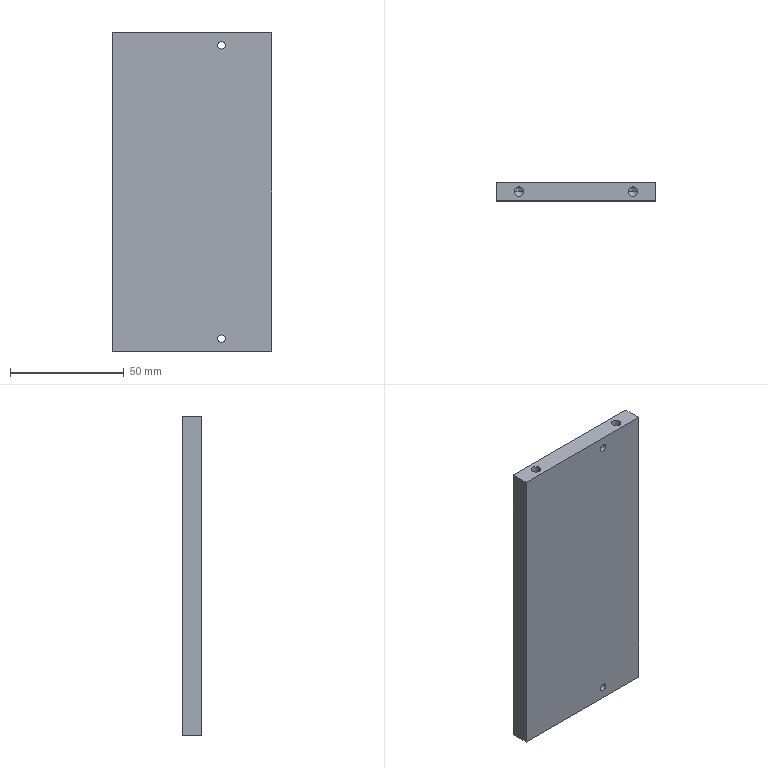Component | SolidWorks | 111.1-1 | 1 solid | 26 faces | box 70 x 8 x 140 mm | volume 77553 mm3 | cylinder 12 | cone 8 | plane 6 | commonest cylinder face diameters 4.2 x8 3.3 x4
build123d program:
from build123d import *

# Parameters (mm, degrees)
SKETCH1_W             = 140
SKETCH1_H             = 70
BOSS_EXTRUDE1_DEPTH   = 8
M5_TAPPED_HOLE1_D     = 4.2
M5_TAPPED_HOLE1_DEPTH = 12.4
M5_TAPPED_HOLE1_TIP   = 1.262
M5_TAPPED_HOLE2_D     = 4.2
M5_TAPPED_HOLE2_DEPTH = 12.4
M5_TAPPED_HOLE2_TIP   = 1.262
M4_TAPPED_HOLE1_D     = 3.3
M4_TAPPED_HOLE1_DEPTH = 10.1
M4_TAPPED_HOLE1_TIP   = 0.9914


with BuildPart() as part:
    # Sketch1 → Boss-Extrude1 (new body)
    with BuildSketch(Plane(origin=(0, 0, 0), x_dir=(1, 0, 0), z_dir=(0, 1, 0))):
        Rectangle(SKETCH1_W, SKETCH1_H)
    extrude(amount=BOSS_EXTRUDE1_DEPTH)

    # M5 Tapped Hole1
    with Locations(Plane(origin=(70, 0, 0), x_dir=(0, 0, -1), z_dir=(1, 0, 0))):
        with Locations((-25, 4), (25, 4)):
            Hole(M5_TAPPED_HOLE1_D / 2, depth=M5_TAPPED_HOLE1_DEPTH)
            with Locations((0, 0, -(M5_TAPPED_HOLE1_DEPTH + M5_TAPPED_HOLE1_TIP / 2))):  # 118° drill point
                Cone(0, M5_TAPPED_HOLE1_D / 2, M5_TAPPED_HOLE1_TIP, mode=Mode.SUBTRACT)

    # M5 Tapped Hole2
    with Locations(Plane.ZY.offset(70)):
        with Locations((-25, 4), (25, 4)):
            Hole(M5_TAPPED_HOLE2_D / 2, depth=M5_TAPPED_HOLE2_DEPTH)
            with Locations((0, 0, -(M5_TAPPED_HOLE2_DEPTH + M5_TAPPED_HOLE2_TIP / 2))):  # 118° drill point
                Cone(0, M5_TAPPED_HOLE2_D / 2, M5_TAPPED_HOLE2_TIP, mode=Mode.SUBTRACT)

    # M4 Tapped Hole1
    with Locations(Plane(origin=(0, 8, 0), x_dir=(-1, 0, 0), z_dir=(0, 1, 0))):
        with Locations((64.5, -13), (-64.5, -13)):
            Hole(M4_TAPPED_HOLE1_D / 2, depth=M4_TAPPED_HOLE1_DEPTH)
            with Locations((0, 0, -(M4_TAPPED_HOLE1_DEPTH + M4_TAPPED_HOLE1_TIP / 2))):  # 118° drill point
                Cone(0, M4_TAPPED_HOLE1_D / 2, M4_TAPPED_HOLE1_TIP, mode=Mode.SUBTRACT)


solid = part.part

# Placed as in the assembly
solid = solid.moved(Location((92, 142, 0), (0, -90, 0)))
STEP:
#1=COLOUR_RGB('',0.7922,0.8196,0.9333);
#2=FILL_AREA_STYLE_COLOUR('',#1);
#3=FILL_AREA_STYLE('',(#2));
#4=SURFACE_STYLE_FILL_AREA(#3);
#5=SURFACE_SIDE_STYLE('',(#4));
#6=SURFACE_STYLE_USAGE(.BOTH.,#5);
#7=PRESENTATION_STYLE_ASSIGNMENT((#6));
#8=CARTESIAN_POINT('',(4.199,5.591,-2.539));
#9=VERTEX_POINT('',#8);
#10=CARTESIAN_POINT('',(4.069,5.591,-2.539));
#11=VERTEX_POINT('',#10);
#12=CARTESIAN_POINT('',(4.134,5.591,-2.539));
#13=DIRECTION('',(0.,1.,0.));
#14=DIRECTION('',(-1.,0.,0.));
#15=AXIS2_PLACEMENT_3D('',#12,#13,#14);
#16=CIRCLE('',#15,0.06496);
#17=EDGE_CURVE('',#9,#11,#16,.T.);
#18=ORIENTED_EDGE('',*,*,#17,.F.);
#19=CARTESIAN_POINT('',(4.199,5.906,-2.539));
#20=VERTEX_POINT('',#19);
#21=CARTESIAN_POINT('',(4.199,5.906,-2.539));
#22=DIRECTION('',(0.,1.,0.));
#23=VECTOR('',#22,39.37);
#24=LINE('',#21,#23);
#25=EDGE_CURVE('',#9,#20,#24,.T.);
#26=ORIENTED_EDGE('',*,*,#25,.T.);
#27=CARTESIAN_POINT('',(4.069,5.906,-2.539));
#28=VERTEX_POINT('',#27);
#29=CARTESIAN_POINT('',(4.134,5.906,-2.539));
#30=DIRECTION('',(0.,1.,0.));
#31=DIRECTION('',(-1.,0.,0.));
#32=AXIS2_PLACEMENT_3D('',#29,#30,#31);
#33=CIRCLE('',#32,0.06496);
#34=EDGE_CURVE('',#20,#28,#33,.T.);
#35=ORIENTED_EDGE('',*,*,#34,.T.);
#36=CARTESIAN_POINT('',(4.069,5.906,-2.539));
#37=DIRECTION('',(0.,1.,0.));
#38=VECTOR('',#37,39.37);
#39=LINE('',#36,#38);
#40=EDGE_CURVE('',#11,#28,#39,.T.);
#41=ORIENTED_EDGE('',*,*,#40,.F.);
#42=EDGE_LOOP('',(#18,#26,#35,#41));
#43=FACE_OUTER_BOUND('',#42,.T.);
#44=CARTESIAN_POINT('',(4.134,5.906,-2.539));
#45=DIRECTION('',(0.,1.,0.));
#46=DIRECTION('',(-1.,0.,0.));
#47=AXIS2_PLACEMENT_3D('',#44,#45,#46);
#48=CYLINDRICAL_SURFACE('',#47,0.06496);
#49=ADVANCED_FACE('',(#43),#48,.F.);
#50=CARTESIAN_POINT('',(4.199,5.591,2.539));
#51=VERTEX_POINT('',#50);
#52=CARTESIAN_POINT('',(4.069,5.591,2.539));
#53=VERTEX_POINT('',#52);
#54=CARTESIAN_POINT('',(4.134,5.591,2.539));
#55=DIRECTION('',(0.,1.,0.));
#56=DIRECTION('',(-1.,0.,0.));
#57=AXIS2_PLACEMENT_3D('',#54,#55,#56);
#58=CIRCLE('',#57,0.06496);
#59=EDGE_CURVE('',#51,#53,#58,.T.);
#60=ORIENTED_EDGE('',*,*,#59,.F.);
#61=CARTESIAN_POINT('',(4.199,5.906,2.539));
#62=VERTEX_POINT('',#61);
#63=CARTESIAN_POINT('',(4.199,5.906,2.539));
#64=DIRECTION('',(0.,1.,0.));
#65=VECTOR('',#64,39.37);
#66=LINE('',#63,#65);
#67=EDGE_CURVE('',#51,#62,#66,.T.);
#68=ORIENTED_EDGE('',*,*,#67,.T.);
#69=CARTESIAN_POINT('',(4.069,5.906,2.539));
#70=VERTEX_POINT('',#69);
#71=CARTESIAN_POINT('',(4.134,5.906,2.539));
#72=DIRECTION('',(0.,1.,0.));
#73=DIRECTION('',(-1.,0.,0.));
#74=AXIS2_PLACEMENT_3D('',#71,#72,#73);
#75=CIRCLE('',#74,0.06496);
#76=EDGE_CURVE('',#62,#70,#75,.T.);
#77=ORIENTED_EDGE('',*,*,#76,.T.);
#78=CARTESIAN_POINT('',(4.069,5.906,2.539));
#79=DIRECTION('',(0.,1.,0.));
#80=VECTOR('',#79,39.37);
#81=LINE('',#78,#80);
#82=EDGE_CURVE('',#53,#70,#81,.T.);
#83=ORIENTED_EDGE('',*,*,#82,.F.);
#84=EDGE_LOOP('',(#60,#68,#77,#83));
#85=FACE_OUTER_BOUND('',#84,.T.);
#86=CARTESIAN_POINT('',(4.134,5.906,2.539));
#87=DIRECTION('',(0.,1.,0.));
#88=DIRECTION('',(-1.,0.,0.));
#89=AXIS2_PLACEMENT_3D('',#86,#87,#88);
#90=CYLINDRICAL_SURFACE('',#89,0.06496);
#91=ADVANCED_FACE('',(#85),#90,.F.);
#92=CARTESIAN_POINT('',(4.689,5.748,-2.268));
#93=VERTEX_POINT('',#92);
#94=CARTESIAN_POINT('',(4.524,5.748,-2.268));
#95=VERTEX_POINT('',#94);
#96=CARTESIAN_POINT('',(4.606,5.748,-2.268));
#97=DIRECTION('',(-0.,0.,-1.));
#98=DIRECTION('',(-1.,0.,0.));
#99=AXIS2_PLACEMENT_3D('',#96,#97,#98);
#100=CIRCLE('',#99,0.08268);
#101=EDGE_CURVE('',#93,#95,#100,.T.);
#102=ORIENTED_EDGE('',*,*,#101,.F.);
#103=CARTESIAN_POINT('',(4.689,5.748,-2.756));
#104=VERTEX_POINT('',#103);
#105=CARTESIAN_POINT('',(4.689,5.748,-2.756));
#106=DIRECTION('',(-0.,0.,-1.));
#107=VECTOR('',#106,39.37);
#108=LINE('',#105,#107);
#109=EDGE_CURVE('',#93,#104,#108,.T.);
#110=ORIENTED_EDGE('',*,*,#109,.T.);
#111=CARTESIAN_POINT('',(4.524,5.748,-2.756));
#112=VERTEX_POINT('',#111);
#113=CARTESIAN_POINT('',(4.606,5.748,-2.756));
#114=DIRECTION('',(-0.,0.,-1.));
#115=DIRECTION('',(-1.,0.,0.));
#116=AXIS2_PLACEMENT_3D('',#113,#114,#115);
#117=CIRCLE('',#116,0.08268);
#118=EDGE_CURVE('',#104,#112,#117,.T.);
#119=ORIENTED_EDGE('',*,*,#118,.T.);
#120=CARTESIAN_POINT('',(4.524,5.748,-2.756));
#121=DIRECTION('',(-0.,0.,-1.));
#122=VECTOR('',#121,39.37);
#123=LINE('',#120,#122);
#124=EDGE_CURVE('',#95,#112,#123,.T.);
#125=ORIENTED_EDGE('',*,*,#124,.F.);
#126=EDGE_LOOP('',(#102,#110,#119,#125));
#127=FACE_OUTER_BOUND('',#126,.T.);
#128=CARTESIAN_POINT('',(4.606,5.748,-2.756));
#129=DIRECTION('',(-0.,0.,-1.));
#130=DIRECTION('',(-1.,0.,0.));
#131=AXIS2_PLACEMENT_3D('',#128,#129,#130);
#132=CYLINDRICAL_SURFACE('',#131,0.08268);
#133=ADVANCED_FACE('',(#127),#132,.F.);
#134=CARTESIAN_POINT('',(4.606,5.748,-2.218));
#135=VERTEX_POINT('',#134);
#136=CARTESIAN_POINT('',(4.524,5.748,-2.268));
#137=DIRECTION('',(-0.8572,0.,-0.515));
#138=VECTOR('',#137,39.37);
#139=LINE('',#136,#138);
#140=EDGE_CURVE('',#135,#95,#139,.T.);
#141=ORIENTED_EDGE('',*,*,#140,.F.);
#142=CARTESIAN_POINT('',(4.689,5.748,-2.268));
#143=DIRECTION('',(0.8572,0.,-0.515));
#144=VECTOR('',#143,39.37);
#145=LINE('',#142,#144);
#146=EDGE_CURVE('',#135,#93,#145,.T.);
#147=ORIENTED_EDGE('',*,*,#146,.T.);
#148=ORIENTED_EDGE('',*,*,#101,.T.);
#149=EDGE_LOOP('',(#141,#147,#148));
#150=FACE_OUTER_BOUND('',#149,.T.);
#151=CARTESIAN_POINT('',(4.606,5.748,-2.268));
#152=DIRECTION('',(-0.,0.,-1.));
#153=DIRECTION('',(-1.,0.,0.));
#154=AXIS2_PLACEMENT_3D('',#151,#152,#153);
#155=CONICAL_SURFACE('',#154,0.08268,1.03);
#156=ADVANCED_FACE('',(#150),#155,.F.);
#157=CARTESIAN_POINT('',(2.72,5.748,-2.268));
#158=VERTEX_POINT('',#157);
#159=CARTESIAN_POINT('',(2.555,5.748,-2.268));
#160=VERTEX_POINT('',#159);
#161=CARTESIAN_POINT('',(2.638,5.748,-2.268));
#162=DIRECTION('',(-0.,0.,-1.));
#163=DIRECTION('',(-1.,0.,0.));
#164=AXIS2_PLACEMENT_3D('',#161,#162,#163);
#165=CIRCLE('',#164,0.08268);
#166=EDGE_CURVE('',#158,#160,#165,.T.);
#167=ORIENTED_EDGE('',*,*,#166,.F.);
#168=CARTESIAN_POINT('',(2.72,5.748,-2.756));
#169=VERTEX_POINT('',#168);
#170=CARTESIAN_POINT('',(2.72,5.748,-2.756));
#171=DIRECTION('',(-0.,0.,-1.));
#172=VECTOR('',#171,39.37);
#173=LINE('',#170,#172);
#174=EDGE_CURVE('',#158,#169,#173,.T.);
#175=ORIENTED_EDGE('',*,*,#174,.T.);
#176=CARTESIAN_POINT('',(2.555,5.748,-2.756));
#177=VERTEX_POINT('',#176);
#178=CARTESIAN_POINT('',(2.638,5.748,-2.756));
#179=DIRECTION('',(-0.,0.,-1.));
#180=DIRECTION('',(-1.,0.,0.));
#181=AXIS2_PLACEMENT_3D('',#178,#179,#180);
#182=CIRCLE('',#181,0.08268);
#183=EDGE_CURVE('',#169,#177,#182,.T.);
#184=ORIENTED_EDGE('',*,*,#183,.T.);
#185=CARTESIAN_POINT('',(2.555,5.748,-2.756));
#186=DIRECTION('',(-0.,0.,-1.));
#187=VECTOR('',#186,39.37);
#188=LINE('',#185,#187);
#189=EDGE_CURVE('',#160,#177,#188,.T.);
#190=ORIENTED_EDGE('',*,*,#189,.F.);
#191=EDGE_LOOP('',(#167,#175,#184,#190));
#192=FACE_OUTER_BOUND('',#191,.T.);
#193=CARTESIAN_POINT('',(2.638,5.748,-2.756));
#194=DIRECTION('',(-0.,0.,-1.));
#195=DIRECTION('',(-1.,0.,0.));
#196=AXIS2_PLACEMENT_3D('',#193,#194,#195);
#197=CYLINDRICAL_SURFACE('',#196,0.08268);
#198=ADVANCED_FACE('',(#192),#197,.F.);
#199=CARTESIAN_POINT('',(2.638,5.748,-2.218));
#200=VERTEX_POINT('',#199);
#201=CARTESIAN_POINT('',(2.555,5.748,-2.268));
#202=DIRECTION('',(-0.8572,0.,-0.515));
#203=VECTOR('',#202,39.37);
#204=LINE('',#201,#203);
#205=EDGE_CURVE('',#200,#160,#204,.T.);
#206=ORIENTED_EDGE('',*,*,#205,.F.);
#207=CARTESIAN_POINT('',(2.72,5.748,-2.268));
#208=DIRECTION('',(0.8572,0.,-0.515));
#209=VECTOR('',#208,39.37);
#210=LINE('',#207,#209);
#211=EDGE_CURVE('',#200,#158,#210,.T.);
#212=ORIENTED_EDGE('',*,*,#211,.T.);
#213=ORIENTED_EDGE('',*,*,#166,.T.);
#214=EDGE_LOOP('',(#206,#212,#213));
#215=FACE_OUTER_BOUND('',#214,.T.);
#216=CARTESIAN_POINT('',(2.638,5.748,-2.268));
#217=DIRECTION('',(-0.,0.,-1.));
#218=DIRECTION('',(-1.,0.,0.));
#219=AXIS2_PLACEMENT_3D('',#216,#217,#218);
#220=CONICAL_SURFACE('',#219,0.08268,1.03);
#221=ADVANCED_FACE('',(#215),#220,.F.);
#222=CARTESIAN_POINT('',(2.555,5.748,2.268));
#223=VERTEX_POINT('',#222);
#224=CARTESIAN_POINT('',(2.72,5.748,2.268));
#225=VERTEX_POINT('',#224);
#226=CARTESIAN_POINT('',(2.638,5.748,2.268));
#227=DIRECTION('',(0.,0.,1.));
#228=DIRECTION('',(1.,0.,0.));
#229=AXIS2_PLACEMENT_3D('',#226,#227,#228);
#230=CIRCLE('',#229,0.08268);
#231=EDGE_CURVE('',#223,#225,#230,.T.);
#232=ORIENTED_EDGE('',*,*,#231,.F.);
#233=CARTESIAN_POINT('',(2.555,5.748,2.756));
#234=VERTEX_POINT('',#233);
#235=CARTESIAN_POINT('',(2.555,5.748,2.756));
#236=DIRECTION('',(0.,0.,1.));
#237=VECTOR('',#236,39.37);
#238=LINE('',#235,#237);
#239=EDGE_CURVE('',#223,#234,#238,.T.);
#240=ORIENTED_EDGE('',*,*,#239,.T.);
#241=CARTESIAN_POINT('',(2.72,5.748,2.756));
#242=VERTEX_POINT('',#241);
#243=CARTESIAN_POINT('',(2.638,5.748,2.756));
#244=DIRECTION('',(0.,0.,1.));
#245=DIRECTION('',(1.,0.,0.));
#246=AXIS2_PLACEMENT_3D('',#243,#244,#245);
#247=CIRCLE('',#246,0.08268);
#248=EDGE_CURVE('',#234,#242,#247,.T.);
#249=ORIENTED_EDGE('',*,*,#248,.T.);
#250=CARTESIAN_POINT('',(2.72,5.748,2.756));
#251=DIRECTION('',(0.,0.,1.));
#252=VECTOR('',#251,39.37);
#253=LINE('',#250,#252);
#254=EDGE_CURVE('',#225,#242,#253,.T.);
#255=ORIENTED_EDGE('',*,*,#254,.F.);
#256=EDGE_LOOP('',(#232,#240,#249,#255));
#257=FACE_OUTER_BOUND('',#256,.T.);
#258=CARTESIAN_POINT('',(2.638,5.748,2.756));
#259=DIRECTION('',(0.,0.,1.));
#260=DIRECTION('',(1.,0.,0.));
#261=AXIS2_PLACEMENT_3D('',#258,#259,#260);
#262=CYLINDRICAL_SURFACE('',#261,0.08268);
#263=ADVANCED_FACE('',(#257),#262,.F.);
#264=CARTESIAN_POINT('',(2.638,5.748,2.218));
#265=VERTEX_POINT('',#264);
#266=CARTESIAN_POINT('',(2.72,5.748,2.268));
#267=DIRECTION('',(0.8572,0.,0.515));
#268=VECTOR('',#267,39.37);
#269=LINE('',#266,#268);
#270=EDGE_CURVE('',#265,#225,#269,.T.);
#271=ORIENTED_EDGE('',*,*,#270,.F.);
#272=CARTESIAN_POINT('',(2.555,5.748,2.268));
#273=DIRECTION('',(-0.8572,0.,0.515));
#274=VECTOR('',#273,39.37);
#275=LINE('',#272,#274);
#276=EDGE_CURVE('',#265,#223,#275,.T.);
#277=ORIENTED_EDGE('',*,*,#276,.T.);
#278=ORIENTED_EDGE('',*,*,#231,.T.);
#279=EDGE_LOOP('',(#271,#277,#278));
#280=FACE_OUTER_BOUND('',#279,.T.);
#281=CARTESIAN_POINT('',(2.638,5.748,2.268));
#282=DIRECTION('',(0.,0.,1.));
#283=DIRECTION('',(1.,0.,0.));
#284=AXIS2_PLACEMENT_3D('',#281,#282,#283);
#285=CONICAL_SURFACE('',#284,0.08268,1.03);
#286=ADVANCED_FACE('',(#280),#285,.F.);
#287=CARTESIAN_POINT('',(4.524,5.748,2.268));
#288=VERTEX_POINT('',#287);
#289=CARTESIAN_POINT('',(4.689,5.748,2.268));
#290=VERTEX_POINT('',#289);
#291=CARTESIAN_POINT('',(4.606,5.748,2.268));
#292=DIRECTION('',(0.,0.,1.));
#293=DIRECTION('',(1.,0.,0.));
#294=AXIS2_PLACEMENT_3D('',#291,#292,#293);
#295=CIRCLE('',#294,0.08268);
#296=EDGE_CURVE('',#288,#290,#295,.T.);
#297=ORIENTED_EDGE('',*,*,#296,.F.);
#298=CARTESIAN_POINT('',(4.524,5.748,2.756));
#299=VERTEX_POINT('',#298);
#300=CARTESIAN_POINT('',(4.524,5.748,2.756));
#301=DIRECTION('',(0.,0.,1.));
#302=VECTOR('',#301,39.37);
#303=LINE('',#300,#302);
#304=EDGE_CURVE('',#288,#299,#303,.T.);
#305=ORIENTED_EDGE('',*,*,#304,.T.);
#306=CARTESIAN_POINT('',(4.689,5.748,2.756));
#307=VERTEX_POINT('',#306);
#308=CARTESIAN_POINT('',(4.606,5.748,2.756));
#309=DIRECTION('',(0.,0.,1.));
#310=DIRECTION('',(1.,0.,0.));
#311=AXIS2_PLACEMENT_3D('',#308,#309,#310);
#312=CIRCLE('',#311,0.08268);
#313=EDGE_CURVE('',#299,#307,#312,.T.);
#314=ORIENTED_EDGE('',*,*,#313,.T.);
#315=CARTESIAN_POINT('',(4.689,5.748,2.756));
#316=DIRECTION('',(0.,0.,1.));
#317=VECTOR('',#316,39.37);
#318=LINE('',#315,#317);
#319=EDGE_CURVE('',#290,#307,#318,.T.);
#320=ORIENTED_EDGE('',*,*,#319,.F.);
#321=EDGE_LOOP('',(#297,#305,#314,#320));
#322=FACE_OUTER_BOUND('',#321,.T.);
#323=CARTESIAN_POINT('',(4.606,5.748,2.756));
#324=DIRECTION('',(0.,0.,1.));
#325=DIRECTION('',(1.,0.,0.));
#326=AXIS2_PLACEMENT_3D('',#323,#324,#325);
#327=CYLINDRICAL_SURFACE('',#326,0.08268);
#328=ADVANCED_FACE('',(#322),#327,.F.);
#329=CARTESIAN_POINT('',(4.606,5.748,2.218));
#330=VERTEX_POINT('',#329);
#331=CARTESIAN_POINT('',(4.689,5.748,2.268));
#332=DIRECTION('',(0.8572,0.,0.515));
#333=VECTOR('',#332,39.37);
#334=LINE('',#331,#333);
#335=EDGE_CURVE('',#330,#290,#334,.T.);
#336=ORIENTED_EDGE('',*,*,#335,.F.);
#337=CARTESIAN_POINT('',(4.524,5.748,2.268));
#338=DIRECTION('',(-0.8572,0.,0.515));
#339=VECTOR('',#338,39.37);
#340=LINE('',#337,#339);
#341=EDGE_CURVE('',#330,#288,#340,.T.);
#342=ORIENTED_EDGE('',*,*,#341,.T.);
#343=ORIENTED_EDGE('',*,*,#296,.T.);
#344=EDGE_LOOP('',(#336,#342,#343));
#345=FACE_OUTER_BOUND('',#344,.T.);
#346=CARTESIAN_POINT('',(4.606,5.748,2.268));
#347=DIRECTION('',(0.,0.,1.));
#348=DIRECTION('',(1.,0.,0.));
#349=AXIS2_PLACEMENT_3D('',#346,#347,#348);
#350=CONICAL_SURFACE('',#349,0.08268,1.03);
#351=ADVANCED_FACE('',(#345),#350,.F.);
#352=CARTESIAN_POINT('',(2.638,5.748,2.756));
#353=DIRECTION('',(0.,0.,1.));
#354=DIRECTION('',(1.,0.,0.));
#355=AXIS2_PLACEMENT_3D('',#352,#353,#354);
#356=CIRCLE('',#355,0.08268);
#357=EDGE_CURVE('',#242,#234,#356,.T.);
#358=ORIENTED_EDGE('',*,*,#357,.F.);
#359=ORIENTED_EDGE('',*,*,#248,.F.);
#360=EDGE_LOOP('',(#358,#359));
#361=FACE_BOUND('',#360,.T.);
#362=CARTESIAN_POINT('',(2.244,5.591,2.756));
#363=VERTEX_POINT('',#362);
#364=CARTESIAN_POINT('',(5.,5.591,2.756));
#365=VERTEX_POINT('',#364);
#366=CARTESIAN_POINT('',(5.,5.591,2.756));
#367=DIRECTION('',(1.,0.,-0.));
#368=VECTOR('',#367,39.37);
#369=LINE('',#366,#368);
#370=EDGE_CURVE('',#363,#365,#369,.T.);
#371=ORIENTED_EDGE('',*,*,#370,.T.);
#372=CARTESIAN_POINT('',(5.,5.906,2.756));
#373=VERTEX_POINT('',#372);
#374=CARTESIAN_POINT('',(5.,5.906,2.756));
#375=DIRECTION('',(0.,-1.,0.));
#376=VECTOR('',#375,39.37);
#377=LINE('',#374,#376);
#378=EDGE_CURVE('',#373,#365,#377,.T.);
#379=ORIENTED_EDGE('',*,*,#378,.F.);
#380=CARTESIAN_POINT('',(2.244,5.906,2.756));
#381=VERTEX_POINT('',#380);
#382=CARTESIAN_POINT('',(5.,5.906,2.756));
#383=DIRECTION('',(1.,0.,-0.));
#384=VECTOR('',#383,39.37);
#385=LINE('',#382,#384);
#386=EDGE_CURVE('',#381,#373,#385,.T.);
#387=ORIENTED_EDGE('',*,*,#386,.F.);
#388=CARTESIAN_POINT('',(2.244,5.906,2.756));
#389=DIRECTION('',(0.,-1.,0.));
#390=VECTOR('',#389,39.37);
#391=LINE('',#388,#390);
#392=EDGE_CURVE('',#381,#363,#391,.T.);
#393=ORIENTED_EDGE('',*,*,#392,.T.);
#394=EDGE_LOOP('',(#371,#379,#387,#393));
#395=FACE_OUTER_BOUND('',#394,.T.);
#396=CARTESIAN_POINT('',(4.606,5.748,2.756));
#397=DIRECTION('',(0.,0.,1.));
#398=DIRECTION('',(1.,0.,0.));
#399=AXIS2_PLACEMENT_3D('',#396,#397,#398);
#400=CIRCLE('',#399,0.08268);
#401=EDGE_CURVE('',#307,#299,#400,.T.);
#402=ORIENTED_EDGE('',*,*,#401,.F.);
#403=ORIENTED_EDGE('',*,*,#313,.F.);
#404=EDGE_LOOP('',(#402,#403));
#405=FACE_BOUND('',#404,.T.);
#406=CARTESIAN_POINT('',(5.,5.906,2.756));
#407=DIRECTION('',(-0.,0.,-1.));
#408=DIRECTION('',(-1.,0.,0.));
#409=AXIS2_PLACEMENT_3D('',#406,#407,#408);
#410=PLANE('',#409);
#411=ADVANCED_FACE('',(#361,#395,#405),#410,.F.);
#412=CARTESIAN_POINT('',(5.,5.591,-2.756));
#413=VERTEX_POINT('',#412);
#414=CARTESIAN_POINT('',(5.,5.591,-2.756));
#415=DIRECTION('',(0.,0.,-1.));
#416=VECTOR('',#415,39.37);
#417=LINE('',#414,#416);
#418=EDGE_CURVE('',#365,#413,#417,.T.);
#419=ORIENTED_EDGE('',*,*,#418,.T.);
#420=CARTESIAN_POINT('',(5.,5.906,-2.756));
#421=VERTEX_POINT('',#420);
#422=CARTESIAN_POINT('',(5.,5.906,-2.756));
#423=DIRECTION('',(0.,-1.,0.));
#424=VECTOR('',#423,39.37);
#425=LINE('',#422,#424);
#426=EDGE_CURVE('',#421,#413,#425,.T.);
#427=ORIENTED_EDGE('',*,*,#426,.F.);
#428=CARTESIAN_POINT('',(5.,5.906,-2.756));
#429=DIRECTION('',(0.,0.,-1.));
#430=VECTOR('',#429,39.37);
#431=LINE('',#428,#430);
#432=EDGE_CURVE('',#373,#421,#431,.T.);
#433=ORIENTED_EDGE('',*,*,#432,.F.);
#434=ORIENTED_EDGE('',*,*,#378,.T.);
#435=EDGE_LOOP('',(#419,#427,#433,#434));
#436=FACE_OUTER_BOUND('',#435,.T.);
#437=CARTESIAN_POINT('',(5.,5.906,-2.756));
#438=DIRECTION('',(-1.,0.,-0.));
#439=DIRECTION('',(-0.,0.,1.));
#440=AXIS2_PLACEMENT_3D('',#437,#438,#439);
#441=PLANE('',#440);
#442=ADVANCED_FACE('',(#436),#441,.F.);
#443=CARTESIAN_POINT('',(4.606,5.748,-2.756));
#444=DIRECTION('',(-0.,0.,-1.));
#445=DIRECTION('',(-1.,0.,0.));
#446=AXIS2_PLACEMENT_3D('',#443,#444,#445);
#447=CIRCLE('',#446,0.08268);
#448=EDGE_CURVE('',#112,#104,#447,.T.);
#449=ORIENTED_EDGE('',*,*,#448,.F.);
#450=ORIENTED_EDGE('',*,*,#118,.F.);
#451=EDGE_LOOP('',(#449,#450));
#452=FACE_BOUND('',#451,.T.);
#453=CARTESIAN_POINT('',(2.638,5.748,-2.756));
#454=DIRECTION('',(-0.,0.,-1.));
#455=DIRECTION('',(-1.,0.,0.));
#456=AXIS2_PLACEMENT_3D('',#453,#454,#455);
#457=CIRCLE('',#456,0.08268);
#458=EDGE_CURVE('',#177,#169,#457,.T.);
#459=ORIENTED_EDGE('',*,*,#458,.F.);
#460=ORIENTED_EDGE('',*,*,#183,.F.);
#461=EDGE_LOOP('',(#459,#460));
#462=FACE_BOUND('',#461,.T.);
#463=CARTESIAN_POINT('',(2.244,5.591,-2.756));
#464=VERTEX_POINT('',#463);
#465=CARTESIAN_POINT('',(5.,5.591,-2.756));
#466=DIRECTION('',(-1.,0.,0.));
#467=VECTOR('',#466,39.37);
#468=LINE('',#465,#467);
#469=EDGE_CURVE('',#413,#464,#468,.T.);
#470=ORIENTED_EDGE('',*,*,#469,.T.);
#471=CARTESIAN_POINT('',(2.244,5.906,-2.756));
#472=VERTEX_POINT('',#471);
#473=CARTESIAN_POINT('',(2.244,5.906,-2.756));
#474=DIRECTION('',(0.,-1.,0.));
#475=VECTOR('',#474,39.37);
#476=LINE('',#473,#475);
#477=EDGE_CURVE('',#472,#464,#476,.T.);
#478=ORIENTED_EDGE('',*,*,#477,.F.);
#479=CARTESIAN_POINT('',(5.,5.906,-2.756));
#480=DIRECTION('',(-1.,0.,0.));
#481=VECTOR('',#480,39.37);
#482=LINE('',#479,#481);
#483=EDGE_CURVE('',#421,#472,#482,.T.);
#484=ORIENTED_EDGE('',*,*,#483,.F.);
#485=ORIENTED_EDGE('',*,*,#426,.T.);
#486=EDGE_LOOP('',(#470,#478,#484,#485));
#487=FACE_OUTER_BOUND('',#486,.T.);
#488=CARTESIAN_POINT('',(5.,5.906,-2.756));
#489=DIRECTION('',(0.,0.,1.));
#490=DIRECTION('',(1.,0.,-0.));
#491=AXIS2_PLACEMENT_3D('',#488,#489,#490);
#492=PLANE('',#491);
#493=ADVANCED_FACE('',(#452,#462,#487),#492,.F.);
#494=CARTESIAN_POINT('',(2.244,5.591,-2.756));
#495=DIRECTION('',(-0.,0.,1.));
#496=VECTOR('',#495,39.37);
#497=LINE('',#494,#496);
#498=EDGE_CURVE('',#464,#363,#497,.T.);
#499=ORIENTED_EDGE('',*,*,#498,.T.);
#500=ORIENTED_EDGE('',*,*,#392,.F.);
#501=CARTESIAN_POINT('',(2.244,5.906,-2.756));
#502=DIRECTION('',(-0.,0.,1.));
#503=VECTOR('',#502,39.37);
#504=LINE('',#501,#503);
#505=EDGE_CURVE('',#472,#381,#504,.T.);
#506=ORIENTED_EDGE('',*,*,#505,.F.);
#507=ORIENTED_EDGE('',*,*,#477,.T.);
#508=EDGE_LOOP('',(#499,#500,#506,#507));
#509=FACE_OUTER_BOUND('',#508,.T.);
#510=CARTESIAN_POINT('',(2.244,5.906,-2.756));
#511=DIRECTION('',(1.,0.,0.));
#512=DIRECTION('',(0.,0.,-1.));
#513=AXIS2_PLACEMENT_3D('',#510,#511,#512);
#514=PLANE('',#513);
#515=ADVANCED_FACE('',(#509),#514,.F.);
#516=CARTESIAN_POINT('',(4.134,5.906,-2.539));
#517=DIRECTION('',(0.,1.,0.));
#518=DIRECTION('',(-1.,0.,0.));
#519=AXIS2_PLACEMENT_3D('',#516,#517,#518);
#520=CIRCLE('',#519,0.06496);
#521=EDGE_CURVE('',#28,#20,#520,.T.);
#522=ORIENTED_EDGE('',*,*,#521,.F.);
#523=ORIENTED_EDGE('',*,*,#34,.F.);
#524=EDGE_LOOP('',(#522,#523));
#525=FACE_BOUND('',#524,.T.);
#526=CARTESIAN_POINT('',(4.134,5.906,2.539));
#527=DIRECTION('',(0.,1.,0.));
#528=DIRECTION('',(-1.,0.,0.));
#529=AXIS2_PLACEMENT_3D('',#526,#527,#528);
#530=CIRCLE('',#529,0.06496);
#531=EDGE_CURVE('',#70,#62,#530,.T.);
#532=ORIENTED_EDGE('',*,*,#531,.F.);
#533=ORIENTED_EDGE('',*,*,#76,.F.);
#534=EDGE_LOOP('',(#532,#533));
#535=FACE_BOUND('',#534,.T.);
#536=ORIENTED_EDGE('',*,*,#386,.T.);
#537=ORIENTED_EDGE('',*,*,#432,.T.);
#538=ORIENTED_EDGE('',*,*,#483,.T.);
#539=ORIENTED_EDGE('',*,*,#505,.T.);
#540=EDGE_LOOP('',(#536,#537,#538,#539));
#541=FACE_OUTER_BOUND('',#540,.T.);
#542=CARTESIAN_POINT('',(2.244,5.906,2.756));
#543=DIRECTION('',(0.,1.,0.));
#544=DIRECTION('',(-1.,0.,-0.));
#545=AXIS2_PLACEMENT_3D('',#542,#543,#544);
#546=PLANE('',#545);
#547=ADVANCED_FACE('',(#525,#535,#541),#546,.T.);
#548=CARTESIAN_POINT('',(4.134,5.591,-2.539));
#549=DIRECTION('',(0.,1.,0.));
#550=DIRECTION('',(-1.,0.,0.));
#551=AXIS2_PLACEMENT_3D('',#548,#549,#550);
#552=CIRCLE('',#551,0.06496);
#553=EDGE_CURVE('',#11,#9,#552,.T.);
#554=ORIENTED_EDGE('',*,*,#553,.T.);
#555=ORIENTED_EDGE('',*,*,#17,.T.);
#556=EDGE_LOOP('',(#554,#555));
#557=FACE_BOUND('',#556,.T.);
#558=CARTESIAN_POINT('',(4.134,5.591,2.539));
#559=DIRECTION('',(0.,1.,0.));
#560=DIRECTION('',(-1.,0.,0.));
#561=AXIS2_PLACEMENT_3D('',#558,#559,#560);
#562=CIRCLE('',#561,0.06496);
#563=EDGE_CURVE('',#53,#51,#562,.T.);
#564=ORIENTED_EDGE('',*,*,#563,.T.);
#565=ORIENTED_EDGE('',*,*,#59,.T.);
#566=EDGE_LOOP('',(#564,#565));
#567=FACE_BOUND('',#566,.T.);
#568=ORIENTED_EDGE('',*,*,#370,.F.);
#569=ORIENTED_EDGE('',*,*,#498,.F.);
#570=ORIENTED_EDGE('',*,*,#469,.F.);
#571=ORIENTED_EDGE('',*,*,#418,.F.);
#572=EDGE_LOOP('',(#568,#569,#570,#571));
#573=FACE_OUTER_BOUND('',#572,.T.);
#574=CARTESIAN_POINT('',(2.244,5.591,2.756));
#575=DIRECTION('',(0.,1.,0.));
#576=DIRECTION('',(-1.,0.,-0.));
#577=AXIS2_PLACEMENT_3D('',#574,#575,#576);
#578=PLANE('',#577);
#579=ADVANCED_FACE('',(#557,#567,#573),#578,.F.);
#580=ORIENTED_EDGE('',*,*,#341,.F.);
#581=ORIENTED_EDGE('',*,*,#335,.T.);
#582=CARTESIAN_POINT('',(4.606,5.748,2.268));
#583=DIRECTION('',(0.,0.,1.));
#584=DIRECTION('',(1.,0.,0.));
#585=AXIS2_PLACEMENT_3D('',#582,#583,#584);
#586=CIRCLE('',#585,0.08268);
#587=EDGE_CURVE('',#290,#288,#586,.T.);
#588=ORIENTED_EDGE('',*,*,#587,.T.);
#589=EDGE_LOOP('',(#580,#581,#588));
#590=FACE_OUTER_BOUND('',#589,.T.);
#591=CARTESIAN_POINT('',(4.606,5.748,2.268));
#592=DIRECTION('',(0.,0.,1.));
#593=DIRECTION('',(1.,0.,0.));
#594=AXIS2_PLACEMENT_3D('',#591,#592,#593);
#595=CONICAL_SURFACE('',#594,0.08268,1.03);
#596=ADVANCED_FACE('',(#590),#595,.F.);
#597=ORIENTED_EDGE('',*,*,#304,.F.);
#598=ORIENTED_EDGE('',*,*,#587,.F.);
#599=ORIENTED_EDGE('',*,*,#319,.T.);
#600=ORIENTED_EDGE('',*,*,#401,.T.);
#601=EDGE_LOOP('',(#597,#598,#599,#600));
#602=FACE_OUTER_BOUND('',#601,.T.);
#603=CARTESIAN_POINT('',(4.606,5.748,2.756));
#604=DIRECTION('',(0.,0.,1.));
#605=DIRECTION('',(1.,0.,0.));
#606=AXIS2_PLACEMENT_3D('',#603,#604,#605);
#607=CYLINDRICAL_SURFACE('',#606,0.08268);
#608=ADVANCED_FACE('',(#602),#607,.F.);
#609=ORIENTED_EDGE('',*,*,#276,.F.);
#610=ORIENTED_EDGE('',*,*,#270,.T.);
#611=CARTESIAN_POINT('',(2.638,5.748,2.268));
#612=DIRECTION('',(0.,0.,1.));
#613=DIRECTION('',(1.,0.,0.));
#614=AXIS2_PLACEMENT_3D('',#611,#612,#613);
#615=CIRCLE('',#614,0.08268);
#616=EDGE_CURVE('',#225,#223,#615,.T.);
#617=ORIENTED_EDGE('',*,*,#616,.T.);
#618=EDGE_LOOP('',(#609,#610,#617));
#619=FACE_OUTER_BOUND('',#618,.T.);
#620=CARTESIAN_POINT('',(2.638,5.748,2.268));
#621=DIRECTION('',(0.,0.,1.));
#622=DIRECTION('',(1.,0.,0.));
#623=AXIS2_PLACEMENT_3D('',#620,#621,#622);
#624=CONICAL_SURFACE('',#623,0.08268,1.03);
#625=ADVANCED_FACE('',(#619),#624,.F.);
#626=ORIENTED_EDGE('',*,*,#239,.F.);
#627=ORIENTED_EDGE('',*,*,#616,.F.);
#628=ORIENTED_EDGE('',*,*,#254,.T.);
#629=ORIENTED_EDGE('',*,*,#357,.T.);
#630=EDGE_LOOP('',(#626,#627,#628,#629));
#631=FACE_OUTER_BOUND('',#630,.T.);
#632=CARTESIAN_POINT('',(2.638,5.748,2.756));
#633=DIRECTION('',(0.,0.,1.));
#634=DIRECTION('',(1.,0.,0.));
#635=AXIS2_PLACEMENT_3D('',#632,#633,#634);
#636=CYLINDRICAL_SURFACE('',#635,0.08268);
#637=ADVANCED_FACE('',(#631),#636,.F.);
#638=ORIENTED_EDGE('',*,*,#211,.F.);
#639=ORIENTED_EDGE('',*,*,#205,.T.);
#640=CARTESIAN_POINT('',(2.638,5.748,-2.268));
#641=DIRECTION('',(-0.,0.,-1.));
#642=DIRECTION('',(-1.,0.,0.));
#643=AXIS2_PLACEMENT_3D('',#640,#641,#642);
#644=CIRCLE('',#643,0.08268);
#645=EDGE_CURVE('',#160,#158,#644,.T.);
#646=ORIENTED_EDGE('',*,*,#645,.T.);
#647=EDGE_LOOP('',(#638,#639,#646));
#648=FACE_OUTER_BOUND('',#647,.T.);
#649=CARTESIAN_POINT('',(2.638,5.748,-2.268));
#650=DIRECTION('',(-0.,0.,-1.));
#651=DIRECTION('',(-1.,0.,0.));
#652=AXIS2_PLACEMENT_3D('',#649,#650,#651);
#653=CONICAL_SURFACE('',#652,0.08268,1.03);
#654=ADVANCED_FACE('',(#648),#653,.F.);
#655=ORIENTED_EDGE('',*,*,#174,.F.);
#656=ORIENTED_EDGE('',*,*,#645,.F.);
#657=ORIENTED_EDGE('',*,*,#189,.T.);
#658=ORIENTED_EDGE('',*,*,#458,.T.);
#659=EDGE_LOOP('',(#655,#656,#657,#658));
#660=FACE_OUTER_BOUND('',#659,.T.);
#661=CARTESIAN_POINT('',(2.638,5.748,-2.756));
#662=DIRECTION('',(-0.,0.,-1.));
#663=DIRECTION('',(-1.,0.,0.));
#664=AXIS2_PLACEMENT_3D('',#661,#662,#663);
#665=CYLINDRICAL_SURFACE('',#664,0.08268);
#666=ADVANCED_FACE('',(#660),#665,.F.);
#667=ORIENTED_EDGE('',*,*,#146,.F.);
#668=ORIENTED_EDGE('',*,*,#140,.T.);
#669=CARTESIAN_POINT('',(4.606,5.748,-2.268));
#670=DIRECTION('',(-0.,0.,-1.));
#671=DIRECTION('',(-1.,0.,0.));
#672=AXIS2_PLACEMENT_3D('',#669,#670,#671);
#673=CIRCLE('',#672,0.08268);
#674=EDGE_CURVE('',#95,#93,#673,.T.);
#675=ORIENTED_EDGE('',*,*,#674,.T.);
#676=EDGE_LOOP('',(#667,#668,#675));
#677=FACE_OUTER_BOUND('',#676,.T.);
#678=CARTESIAN_POINT('',(4.606,5.748,-2.268));
#679=DIRECTION('',(-0.,0.,-1.));
#680=DIRECTION('',(-1.,0.,0.));
#681=AXIS2_PLACEMENT_3D('',#678,#679,#680);
#682=CONICAL_SURFACE('',#681,0.08268,1.03);
#683=ADVANCED_FACE('',(#677),#682,.F.);
#684=ORIENTED_EDGE('',*,*,#109,.F.);
#685=ORIENTED_EDGE('',*,*,#674,.F.);
#686=ORIENTED_EDGE('',*,*,#124,.T.);
#687=ORIENTED_EDGE('',*,*,#448,.T.);
#688=EDGE_LOOP('',(#684,#685,#686,#687));
#689=FACE_OUTER_BOUND('',#688,.T.);
#690=CARTESIAN_POINT('',(4.606,5.748,-2.756));
#691=DIRECTION('',(-0.,0.,-1.));
#692=DIRECTION('',(-1.,0.,0.));
#693=AXIS2_PLACEMENT_3D('',#690,#691,#692);
#694=CYLINDRICAL_SURFACE('',#693,0.08268);
#695=ADVANCED_FACE('',(#689),#694,.F.);
#696=ORIENTED_EDGE('',*,*,#67,.F.);
#697=ORIENTED_EDGE('',*,*,#563,.F.);
#698=ORIENTED_EDGE('',*,*,#82,.T.);
#699=ORIENTED_EDGE('',*,*,#531,.T.);
#700=EDGE_LOOP('',(#696,#697,#698,#699));
#701=FACE_OUTER_BOUND('',#700,.T.);
#702=CARTESIAN_POINT('',(4.134,5.906,2.539));
#703=DIRECTION('',(0.,1.,0.));
#704=DIRECTION('',(-1.,0.,0.));
#705=AXIS2_PLACEMENT_3D('',#702,#703,#704);
#706=CYLINDRICAL_SURFACE('',#705,0.06496);
#707=ADVANCED_FACE('',(#701),#706,.F.);
#708=ORIENTED_EDGE('',*,*,#25,.F.);
#709=ORIENTED_EDGE('',*,*,#553,.F.);
#710=ORIENTED_EDGE('',*,*,#40,.T.);
#711=ORIENTED_EDGE('',*,*,#521,.T.);
#712=EDGE_LOOP('',(#708,#709,#710,#711));
#713=FACE_OUTER_BOUND('',#712,.T.);
#714=CARTESIAN_POINT('',(4.134,5.906,-2.539));
#715=DIRECTION('',(0.,1.,0.));
#716=DIRECTION('',(-1.,0.,0.));
#717=AXIS2_PLACEMENT_3D('',#714,#715,#716);
#718=CYLINDRICAL_SURFACE('',#717,0.06496);
#719=ADVANCED_FACE('',(#713),#718,.F.);
#720=CLOSED_SHELL('',(#49,#91,#133,#156,#198,#221,#263,#286,#328,#351,#411,#442,#493,#515,#547,#579,#596,#608,#625,#637,#654,#666,#683,#695,#707,#719));
#721=MANIFOLD_SOLID_BREP('',#720);
#722=STYLED_ITEM('',(#7),#721);
#723=PRESENTATION_LAYER_ASSIGNMENT('','',(#722));
#724=CARTESIAN_POINT('',(0.,0.,0.));
#725=DIRECTION('',(0.,0.,1.));
#726=DIRECTION('',(1.,0.,0.));
#727=AXIS2_PLACEMENT_3D('',#724,#725,#726);
#728=(LENGTH_UNIT()NAMED_UNIT(*)SI_UNIT($,.METRE.));
#729=LENGTH_MEASURE_WITH_UNIT(LENGTH_MEASURE(0.0254),#728);
#730=DIMENSIONAL_EXPONENTS(1.,0.,0.,0.,0.,0.,0.);
#731=(CONVERSION_BASED_UNIT('',#729)LENGTH_UNIT()NAMED_UNIT(#730));
#732=UNCERTAINTY_MEASURE_WITH_UNIT(LENGTH_MEASURE(0.00001),#731,'','');
#733=(NAMED_UNIT(*)PLANE_ANGLE_UNIT()SI_UNIT($,.RADIAN.));
#734=(NAMED_UNIT(*)SI_UNIT($,.STERADIAN.)SOLID_ANGLE_UNIT());
#735=(GEOMETRIC_REPRESENTATION_CONTEXT(3)GLOBAL_UNCERTAINTY_ASSIGNED_CONTEXT((#732))GLOBAL_UNIT_ASSIGNED_CONTEXT((#731,#733,#734))REPRESENTATION_CONTEXT('',''));
#736=ADVANCED_BREP_SHAPE_REPRESENTATION('',(#721,#727),#735);
#737=(LENGTH_UNIT()NAMED_UNIT(*)SI_UNIT($,.METRE.));
#738=LENGTH_MEASURE_WITH_UNIT(LENGTH_MEASURE(0.0254),#737);
#739=DIMENSIONAL_EXPONENTS(1.,0.,0.,0.,0.,0.,0.);
#740=(CONVERSION_BASED_UNIT('',#738)LENGTH_UNIT()NAMED_UNIT(#739));
#741=UNCERTAINTY_MEASURE_WITH_UNIT(LENGTH_MEASURE(0.00001),#740,'','');
#742=(NAMED_UNIT(*)PLANE_ANGLE_UNIT()SI_UNIT($,.RADIAN.));
#743=(NAMED_UNIT(*)SI_UNIT($,.STERADIAN.)SOLID_ANGLE_UNIT());
#744=(GEOMETRIC_REPRESENTATION_CONTEXT(3)GLOBAL_UNCERTAINTY_ASSIGNED_CONTEXT((#741))GLOBAL_UNIT_ASSIGNED_CONTEXT((#740,#742,#743))REPRESENTATION_CONTEXT('',''));
#745=MECHANICAL_DESIGN_GEOMETRIC_PRESENTATION_REPRESENTATION('',(#722),#744);